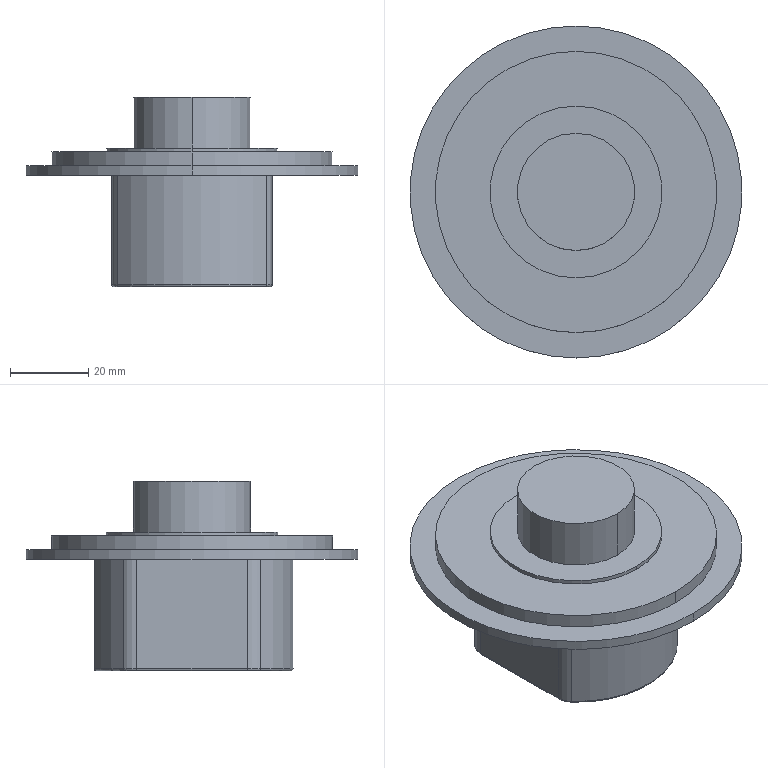Component | SolidWorks | 12AInnerSideWheel-EngravingAndMillingAxis-1_12AInnerSideWheelAxis-2 | 1 solid | 51 faces | volume 84617 mm3 | cylinder 27 | plane 13 | torus 7 | cone 4 | commonest cylinder face diameters 52 x5 10.2 x4 10 x4 8.5 x2 12.5 x2 85 x2 72 x2 44 x2 | material Cr12MoV